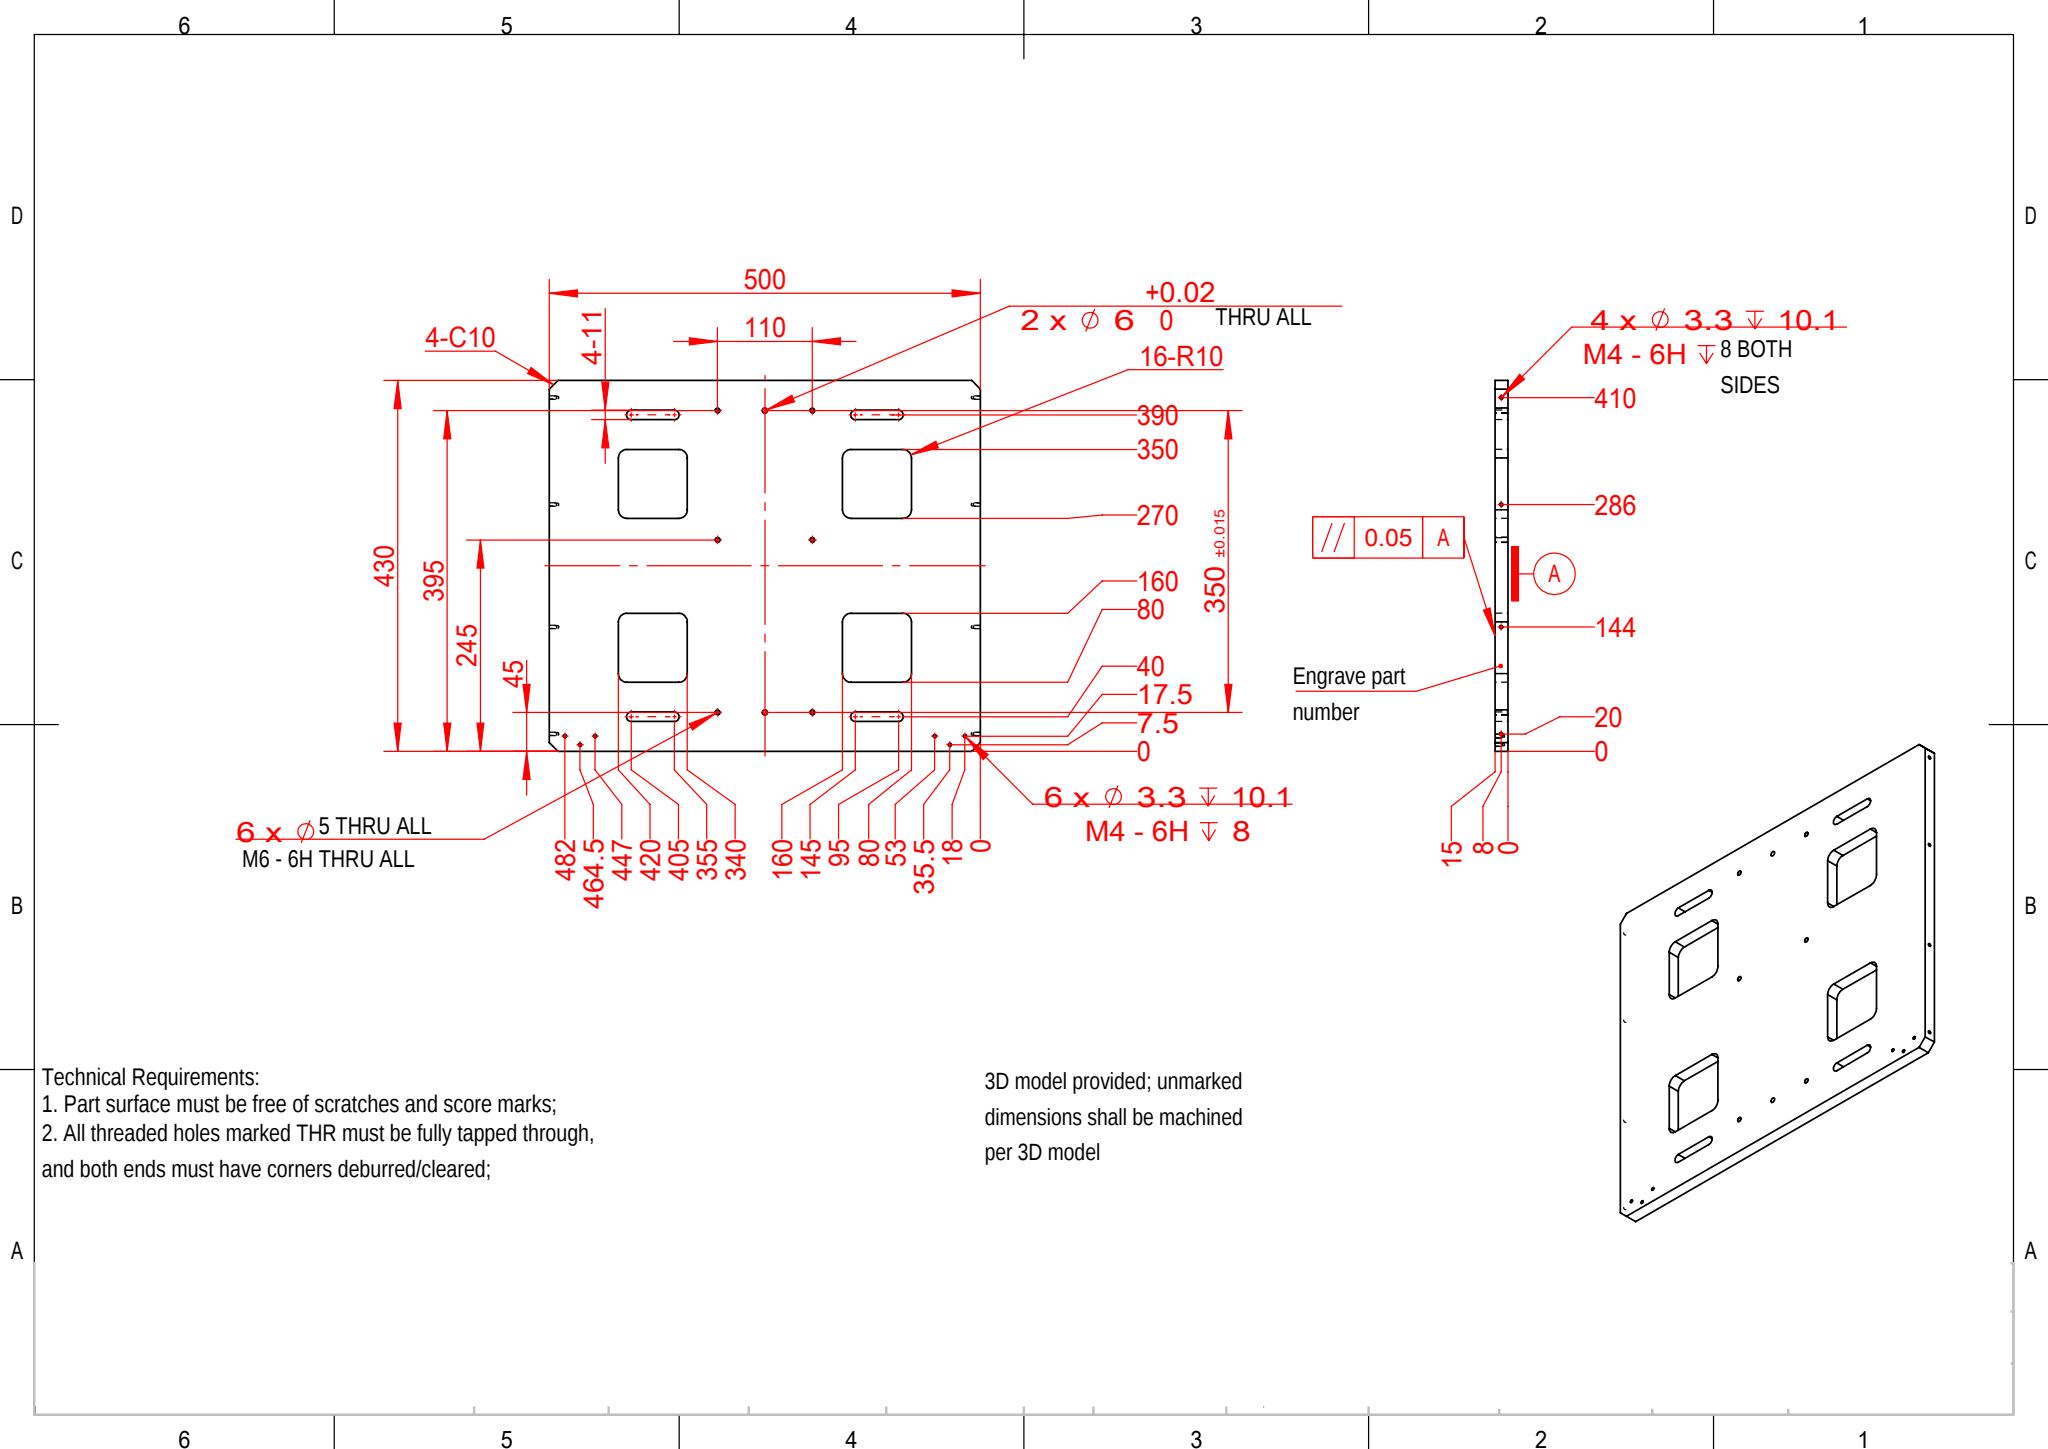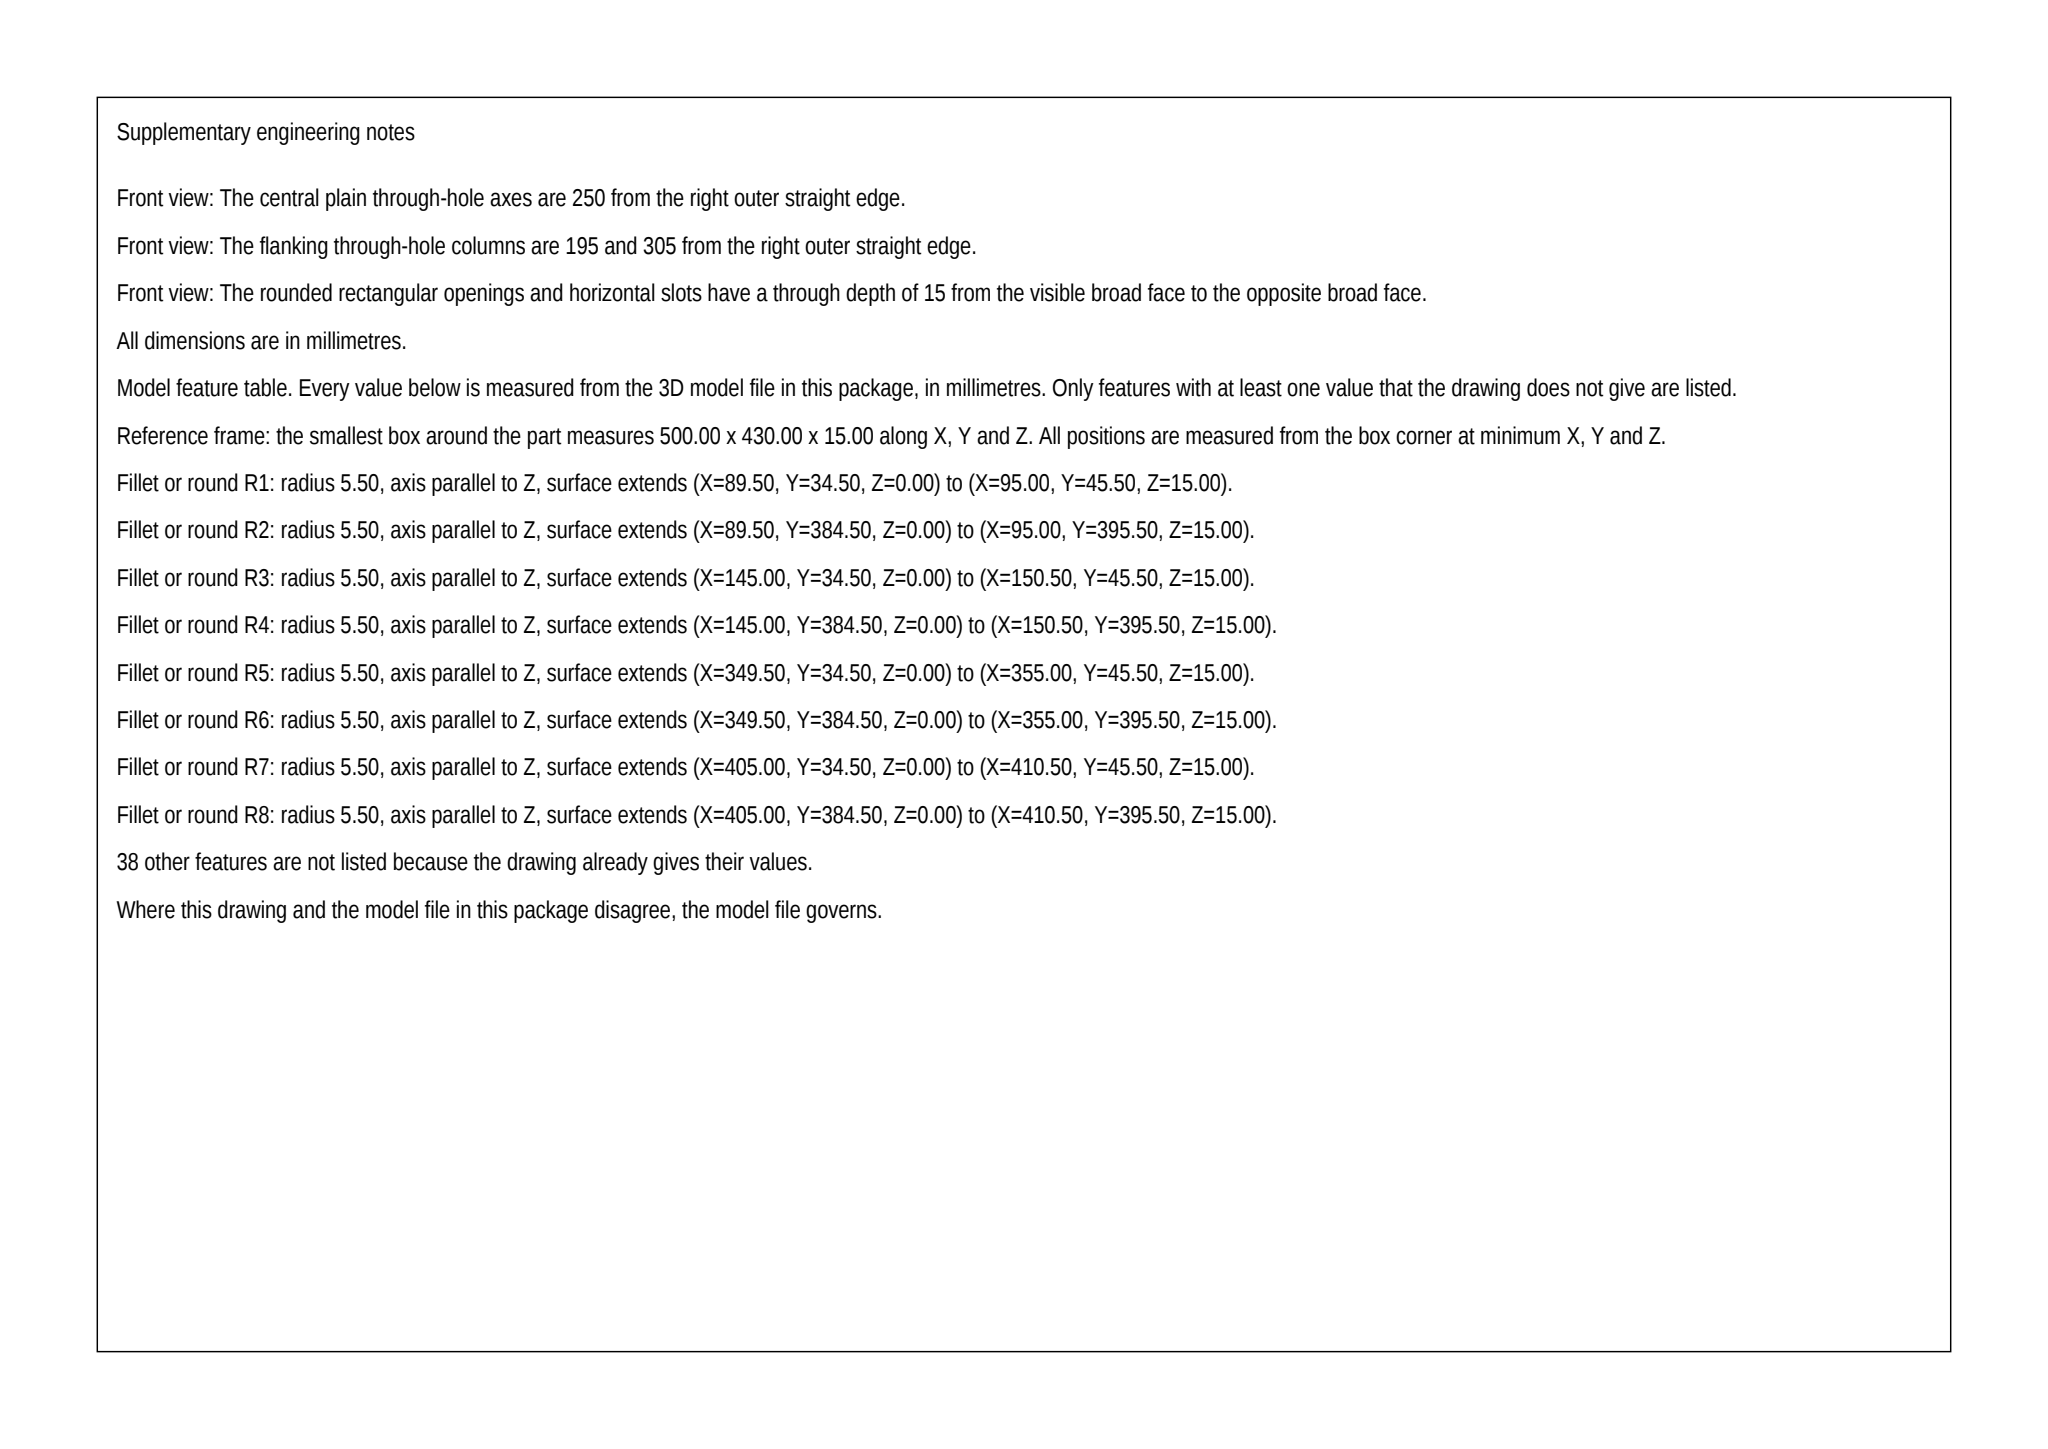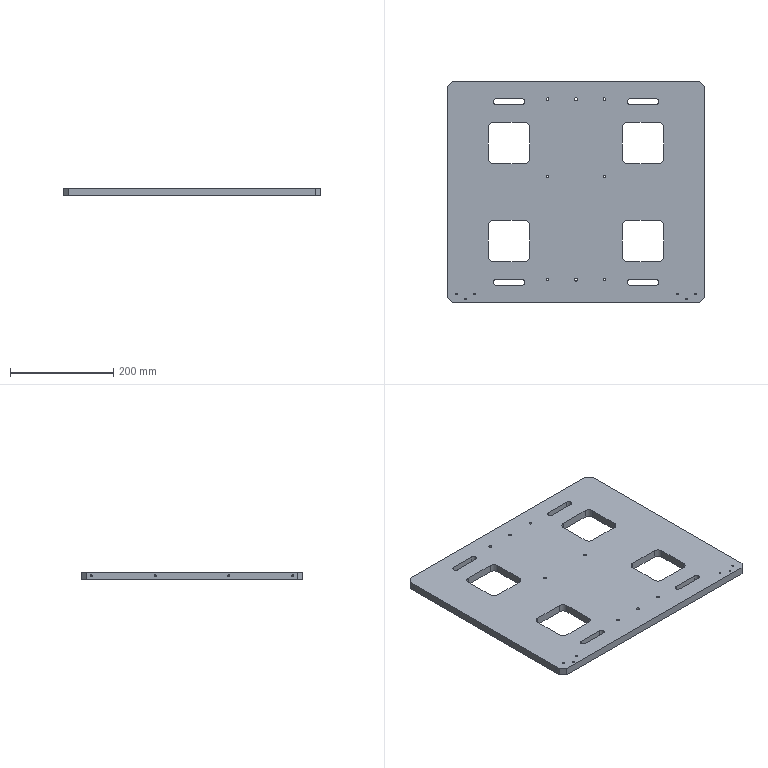Part | SolidWorks | mm | 1 solid | 134 faces | box 500 x 430 x 15 mm | volume 2800584 mm3 | cylinder 72 | plane 34 | cone 28 | commonest cylinder face diameters 3.3 x28 20 x16 11 x12 5 x12 6 x4